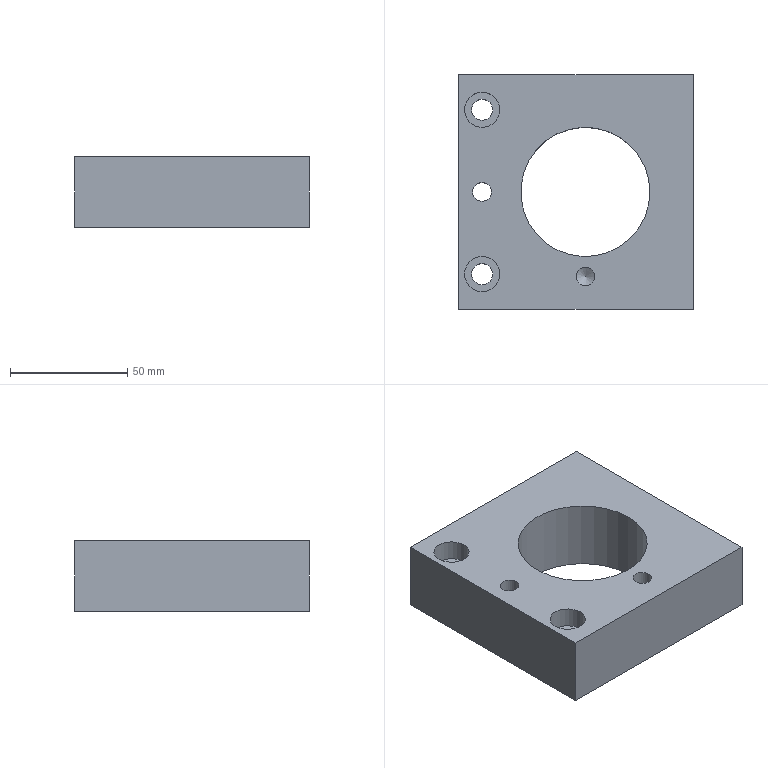Component | NX | BORING_TEMPLATE | 1 solid | 16 faces | volume 220583 mm3 | plane 8 | cylinder 7 | cone 1 | commonest cylinder face diameters 8 x2 9 x2 15 x2 55 x1